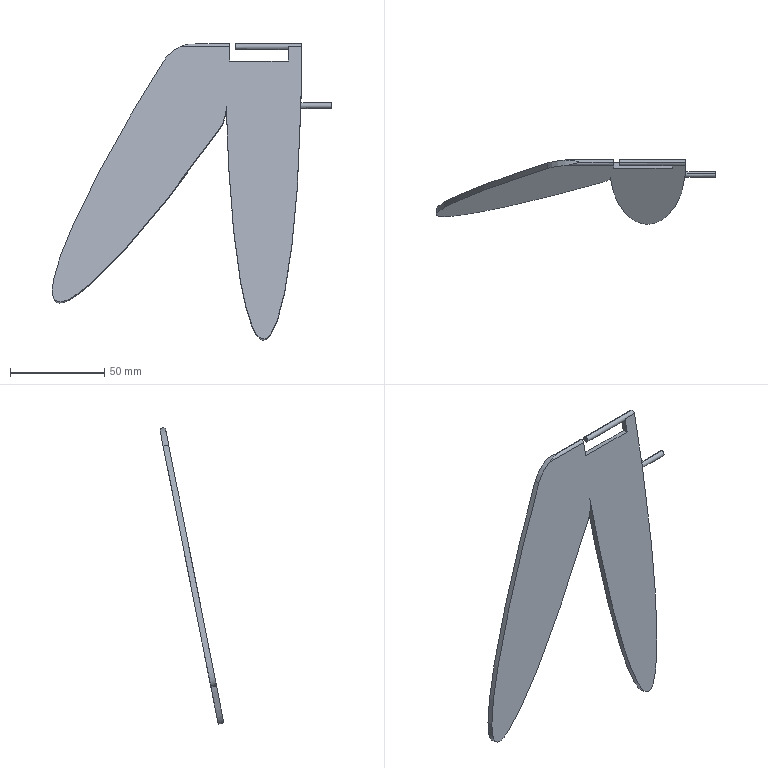Component | SolidWorks | 11-1 | 1 solid | 21 faces | box 147.82 x 33.71 x 156.77 mm | volume 30727 mm3 | cylinder 9 | plane 8 | spline 4 | commonest cylinder face diameters 3 x6 40 x3
STEP:
#1=CARTESIAN_POINT('',(1.359,2.476,-2.286));
#2=VERTEX_POINT('',#1);
#3=CARTESIAN_POINT('',(1.359,2.472,-2.304));
#4=VERTEX_POINT('',#3);
#5=CARTESIAN_POINT('',(0.5717,2.472,-2.304));
#6=DIRECTION('',(-0.,0.9809,-0.1945));
#7=DIRECTION('',(1.,0.,0.));
#8=AXIS2_PLACEMENT_3D('',#5,#6,#7);
#9=CIRCLE('',#8,0.7874);
#10=EDGE_CURVE('',#2,#4,#9,.T.);
#11=ORIENTED_EDGE('',*,*,#10,.T.);
#12=CARTESIAN_POINT('',(1.359,2.588,-2.327));
#13=VERTEX_POINT('',#12);
#14=CARTESIAN_POINT('',(1.359,2.472,-2.304));
#15=DIRECTION('',(-0.,0.9809,-0.1945));
#16=VECTOR('',#15,39.37);
#17=LINE('',#14,#16);
#18=EDGE_CURVE('',#4,#13,#17,.T.);
#19=ORIENTED_EDGE('',*,*,#18,.T.);
#20=CARTESIAN_POINT('',(1.359,2.592,-2.309));
#21=VERTEX_POINT('',#20);
#22=CARTESIAN_POINT('',(0.5717,2.588,-2.327));
#23=DIRECTION('',(-0.,0.9809,-0.1945));
#24=DIRECTION('',(1.,0.,0.));
#25=AXIS2_PLACEMENT_3D('',#22,#23,#24);
#26=CIRCLE('',#25,0.7874);
#27=EDGE_CURVE('',#21,#13,#26,.T.);
#28=ORIENTED_EDGE('',*,*,#27,.F.);
#29=CARTESIAN_POINT('',(1.359,2.476,-2.286));
#30=DIRECTION('',(-0.,0.9809,-0.1945));
#31=VECTOR('',#30,39.37);
#32=LINE('',#29,#31);
#33=EDGE_CURVE('',#2,#21,#32,.T.);
#34=ORIENTED_EDGE('',*,*,#33,.F.);
#35=EDGE_LOOP('',(#11,#19,#28,#34));
#36=FACE_OUTER_BOUND('',#35,.T.);
#37=CARTESIAN_POINT('',(0.5717,2.472,-2.304));
#38=DIRECTION('',(-0.,0.9809,-0.1945));
#39=DIRECTION('',(1.,0.,0.));
#40=AXIS2_PLACEMENT_3D('',#37,#38,#39);
#41=CYLINDRICAL_SURFACE('',#40,0.7874);
#42=ADVANCED_FACE('',(#36),#41,.T.);
#43=CARTESIAN_POINT('',(1.218,2.385,-2.745));
#44=VERTEX_POINT('',#43);
#45=CARTESIAN_POINT('',(-2.187,1.672,-6.337));
#46=VERTEX_POINT('',#45);
#47=CARTESIAN_POINT('',(1.218,2.385,-2.745));
#48=CARTESIAN_POINT('',(-0.5057,1.903,-5.172));
#49=CARTESIAN_POINT('',(-1.827,1.627,-6.566));
#50=CARTESIAN_POINT('',(-2.187,1.672,-6.337));
#51=(BOUNDED_CURVE()B_SPLINE_CURVE(3,(#47,#48,#49,#50),.UNSPECIFIED.,.F.,.T.)B_SPLINE_CURVE_WITH_KNOTS((4,4),(4.959,6.283),.UNSPECIFIED.)CURVE()GEOMETRIC_REPRESENTATION_ITEM()RATIONAL_B_SPLINE_CURVE((1.,0.8591,0.8591,1.))REPRESENTATION_ITEM(''));
#52=EDGE_CURVE('',#44,#46,#51,.T.);
#53=ORIENTED_EDGE('',*,*,#52,.T.);
#54=CARTESIAN_POINT('',(-2.187,1.788,-6.36));
#55=VERTEX_POINT('',#54);
#56=CARTESIAN_POINT('',(-2.187,1.672,-6.337));
#57=DIRECTION('',(-0.,0.9809,-0.1945));
#58=VECTOR('',#57,39.37);
#59=LINE('',#56,#58);
#60=EDGE_CURVE('',#46,#55,#59,.T.);
#61=ORIENTED_EDGE('',*,*,#60,.T.);
#62=CARTESIAN_POINT('',(1.218,2.501,-2.768));
#63=VERTEX_POINT('',#62);
#64=CARTESIAN_POINT('',(1.218,2.501,-2.768));
#65=CARTESIAN_POINT('',(-0.5057,2.019,-5.195));
#66=CARTESIAN_POINT('',(-1.827,1.743,-6.589));
#67=CARTESIAN_POINT('',(-2.187,1.788,-6.36));
#68=(BOUNDED_CURVE()B_SPLINE_CURVE(3,(#64,#65,#66,#67),.UNSPECIFIED.,.F.,.T.)B_SPLINE_CURVE_WITH_KNOTS((4,4),(4.959,6.283),.UNSPECIFIED.)CURVE()GEOMETRIC_REPRESENTATION_ITEM()RATIONAL_B_SPLINE_CURVE((1.,0.8591,0.8591,1.))REPRESENTATION_ITEM(''));
#69=EDGE_CURVE('',#63,#55,#68,.T.);
#70=ORIENTED_EDGE('',*,*,#69,.F.);
#71=CARTESIAN_POINT('',(1.218,2.385,-2.745));
#72=DIRECTION('',(-0.,0.9809,-0.1945));
#73=VECTOR('',#72,39.37);
#74=LINE('',#71,#73);
#75=EDGE_CURVE('',#44,#63,#74,.T.);
#76=ORIENTED_EDGE('',*,*,#75,.F.);
#77=EDGE_LOOP('',(#53,#61,#70,#76));
#78=FACE_OUTER_BOUND('',#77,.T.);
#79=CARTESIAN_POINT('',(1.218,2.385,-2.745));
#80=CARTESIAN_POINT('',(1.218,2.501,-2.768));
#81=CARTESIAN_POINT('',(-0.5057,1.903,-5.172));
#82=CARTESIAN_POINT('',(-0.5057,2.019,-5.195));
#83=CARTESIAN_POINT('',(-1.827,1.627,-6.566));
#84=CARTESIAN_POINT('',(-1.827,1.743,-6.589));
#85=CARTESIAN_POINT('',(-2.187,1.672,-6.337));
#86=CARTESIAN_POINT('',(-2.187,1.788,-6.36));
#87=(BOUNDED_SURFACE()B_SPLINE_SURFACE(3,1,((#79,#80),(#81,#82),(#83,#84),(#85,#86)),.UNSPECIFIED.,.F.,.F.,.T.)B_SPLINE_SURFACE_WITH_KNOTS((4,4),(2,2),(0.,1.),(0.,1.),.UNSPECIFIED.)GEOMETRIC_REPRESENTATION_ITEM()RATIONAL_B_SPLINE_SURFACE(((1.,1.),(0.8591,0.8591),(0.8591,0.8591),(1.,1.)))REPRESENTATION_ITEM('')SURFACE());
#88=ADVANCED_FACE('',(#78),#87,.T.);
#89=CARTESIAN_POINT('',(3.553,2.528,-2.328));
#90=VERTEX_POINT('',#89);
#91=CARTESIAN_POINT('',(3.553,2.551,-2.212));
#92=VERTEX_POINT('',#91);
#93=CARTESIAN_POINT('',(3.553,2.539,-2.27));
#94=DIRECTION('',(1.,0.,0.));
#95=DIRECTION('',(0.,-0.1945,-0.9809));
#96=AXIS2_PLACEMENT_3D('',#93,#94,#95);
#97=CIRCLE('',#96,0.05906);
#98=EDGE_CURVE('',#90,#92,#97,.T.);
#99=ORIENTED_EDGE('',*,*,#98,.F.);
#100=CARTESIAN_POINT('',(2.912,2.528,-2.328));
#101=VERTEX_POINT('',#100);
#102=CARTESIAN_POINT('',(3.553,2.528,-2.328));
#103=DIRECTION('',(-1.,-0.,-0.));
#104=VECTOR('',#103,39.37);
#105=LINE('',#102,#104);
#106=EDGE_CURVE('',#90,#101,#105,.T.);
#107=ORIENTED_EDGE('',*,*,#106,.T.);
#108=CARTESIAN_POINT('',(2.913,2.597,-2.282));
#109=VERTEX_POINT('',#108);
#110=CARTESIAN_POINT('',(2.913,2.597,-2.282));
#111=CARTESIAN_POINT('',(2.913,2.596,-2.289));
#112=CARTESIAN_POINT('',(2.913,2.592,-2.297));
#113=CARTESIAN_POINT('',(2.912,2.584,-2.309));
#114=CARTESIAN_POINT('',(2.912,2.578,-2.315));
#115=CARTESIAN_POINT('',(2.912,2.569,-2.322));
#116=CARTESIAN_POINT('',(2.912,2.565,-2.323));
#117=CARTESIAN_POINT('',(2.912,2.558,-2.326));
#118=CARTESIAN_POINT('',(2.912,2.554,-2.327));
#119=CARTESIAN_POINT('',(2.912,2.547,-2.329));
#120=CARTESIAN_POINT('',(2.912,2.543,-2.329));
#121=CARTESIAN_POINT('',(2.912,2.535,-2.329));
#122=CARTESIAN_POINT('',(2.912,2.531,-2.329));
#123=CARTESIAN_POINT('',(2.912,2.528,-2.328));
#124=B_SPLINE_CURVE_WITH_KNOTS('',3,(#110,#111,#112,#113,#114,#115,#116,#117,#118,#119,#120,#121,#122,#123),.UNSPECIFIED.,.F.,.F.,(4,2,2,2,2,2,4),(0.00469,0.005277,0.005863,0.006156,0.00645,0.006743,0.007036),.UNSPECIFIED.);
#125=EDGE_CURVE('',#109,#101,#124,.T.);
#126=ORIENTED_EDGE('',*,*,#125,.F.);
#127=CARTESIAN_POINT('',(2.914,2.551,-2.212));
#128=VERTEX_POINT('',#127);
#129=CARTESIAN_POINT('',(2.914,2.551,-2.212));
#130=CARTESIAN_POINT('',(2.914,2.554,-2.213));
#131=CARTESIAN_POINT('',(2.914,2.558,-2.214));
#132=CARTESIAN_POINT('',(2.914,2.565,-2.217));
#133=CARTESIAN_POINT('',(2.914,2.569,-2.219));
#134=CARTESIAN_POINT('',(2.914,2.575,-2.223));
#135=CARTESIAN_POINT('',(2.914,2.578,-2.226));
#136=CARTESIAN_POINT('',(2.914,2.584,-2.231));
#137=CARTESIAN_POINT('',(2.914,2.586,-2.234));
#138=CARTESIAN_POINT('',(2.914,2.592,-2.244));
#139=CARTESIAN_POINT('',(2.914,2.595,-2.251));
#140=CARTESIAN_POINT('',(2.914,2.598,-2.263));
#141=CARTESIAN_POINT('',(2.913,2.598,-2.266));
#142=CARTESIAN_POINT('',(2.913,2.598,-2.274));
#143=CARTESIAN_POINT('',(2.913,2.598,-2.278));
#144=CARTESIAN_POINT('',(2.913,2.597,-2.282));
#145=B_SPLINE_CURVE_WITH_KNOTS('',3,(#129,#130,#131,#132,#133,#134,#135,#136,#137,#138,#139,#140,#141,#142,#143,#144),.UNSPECIFIED.,.F.,.F.,(4,2,2,2,2,2,2,4),(0.002346,0.002639,0.002932,0.003225,0.003518,0.004104,0.004397,0.00469),.UNSPECIFIED.);
#146=EDGE_CURVE('',#128,#109,#145,.T.);
#147=ORIENTED_EDGE('',*,*,#146,.F.);
#148=CARTESIAN_POINT('',(3.553,2.551,-2.212));
#149=DIRECTION('',(-1.,-0.,-0.));
#150=VECTOR('',#149,39.37);
#151=LINE('',#148,#150);
#152=EDGE_CURVE('',#92,#128,#151,.T.);
#153=ORIENTED_EDGE('',*,*,#152,.F.);
#154=EDGE_LOOP('',(#99,#107,#126,#147,#153));
#155=FACE_OUTER_BOUND('',#154,.T.);
#156=CARTESIAN_POINT('',(3.553,2.539,-2.27));
#157=DIRECTION('',(-1.,-0.,-0.));
#158=DIRECTION('',(0.,0.1945,0.9809));
#159=AXIS2_PLACEMENT_3D('',#156,#157,#158);
#160=CYLINDRICAL_SURFACE('',#159,0.05906);
#161=ADVANCED_FACE('',(#155),#160,.T.);
#162=CARTESIAN_POINT('',(1.427,2.794,-0.9829));
#163=VERTEX_POINT('',#162);
#164=CARTESIAN_POINT('',(1.427,2.725,-1.029));
#165=VERTEX_POINT('',#164);
#166=CARTESIAN_POINT('',(1.427,2.783,-1.041));
#167=DIRECTION('',(1.,0.,0.));
#168=DIRECTION('',(0.,-0.1945,-0.9809));
#169=AXIS2_PLACEMENT_3D('',#166,#167,#168);
#170=CIRCLE('',#169,0.05906);
#171=EDGE_CURVE('',#163,#165,#170,.T.);
#172=ORIENTED_EDGE('',*,*,#171,.F.);
#173=CARTESIAN_POINT('',(0.7196,2.794,-0.9829));
#174=VERTEX_POINT('',#173);
#175=CARTESIAN_POINT('',(2.923,2.794,-0.9829));
#176=DIRECTION('',(-1.,-0.,-0.));
#177=VECTOR('',#176,39.37);
#178=LINE('',#175,#177);
#179=EDGE_CURVE('',#163,#174,#178,.T.);
#180=ORIENTED_EDGE('',*,*,#179,.T.);
#181=CARTESIAN_POINT('',(0.4204,2.725,-1.029));
#182=VERTEX_POINT('',#181);
#183=CARTESIAN_POINT('',(0.7196,2.794,-0.9829));
#184=CARTESIAN_POINT('',(0.7071,2.791,-0.9823));
#185=CARTESIAN_POINT('',(0.6944,2.788,-0.9819));
#186=CARTESIAN_POINT('',(0.6692,2.781,-0.9818));
#187=CARTESIAN_POINT('',(0.6567,2.777,-0.982));
#188=CARTESIAN_POINT('',(0.619,2.767,-0.9836));
#189=CARTESIAN_POINT('',(0.594,2.76,-0.986));
#190=CARTESIAN_POINT('',(0.544,2.747,-0.9934));
#191=CARTESIAN_POINT('',(0.5188,2.741,-0.9984));
#192=CARTESIAN_POINT('',(0.4693,2.731,-1.012));
#193=CARTESIAN_POINT('',(0.4448,2.727,-1.02));
#194=CARTESIAN_POINT('',(0.4204,2.725,-1.029));
#195=B_SPLINE_CURVE_WITH_KNOTS('',3,(#183,#184,#185,#186,#187,#188,#189,#190,#191,#192,#193,#194),.UNSPECIFIED.,.F.,.F.,(4,2,2,2,2,4),(-0.00002828,0.0009634,0.001955,0.003939,0.005922,0.007905),.UNSPECIFIED.);
#196=EDGE_CURVE('',#174,#182,#195,.T.);
#197=ORIENTED_EDGE('',*,*,#196,.T.);
#198=CARTESIAN_POINT('',(1.348,2.725,-1.029));
#199=DIRECTION('',(1.,0.,0.));
#200=VECTOR('',#199,39.37);
#201=LINE('',#198,#200);
#202=EDGE_CURVE('',#182,#165,#201,.T.);
#203=ORIENTED_EDGE('',*,*,#202,.T.);
#204=EDGE_LOOP('',(#172,#180,#197,#203));
#205=FACE_OUTER_BOUND('',#204,.T.);
#206=CARTESIAN_POINT('',(2.923,2.783,-1.041));
#207=DIRECTION('',(-1.,-0.,-0.));
#208=DIRECTION('',(0.,0.1945,0.9809));
#209=AXIS2_PLACEMENT_3D('',#206,#207,#208);
#210=CYLINDRICAL_SURFACE('',#209,0.05906);
#211=ADVANCED_FACE('',(#205),#210,.T.);
#212=CARTESIAN_POINT('',(2.648,2.771,-1.099));
#213=VERTEX_POINT('',#212);
#214=CARTESIAN_POINT('',(2.648,2.841,-1.052));
#215=VERTEX_POINT('',#214);
#216=CARTESIAN_POINT('',(2.648,2.783,-1.041));
#217=DIRECTION('',(1.,0.,0.));
#218=DIRECTION('',(0.,0.1945,0.9809));
#219=AXIS2_PLACEMENT_3D('',#216,#217,#218);
#220=CIRCLE('',#219,0.05906);
#221=EDGE_CURVE('',#213,#215,#220,.T.);
#222=ORIENTED_EDGE('',*,*,#221,.F.);
#223=CARTESIAN_POINT('',(1.545,2.771,-1.099));
#224=VERTEX_POINT('',#223);
#225=CARTESIAN_POINT('',(2.923,2.771,-1.099));
#226=DIRECTION('',(-1.,-0.,-0.));
#227=VECTOR('',#226,39.37);
#228=LINE('',#225,#227);
#229=EDGE_CURVE('',#213,#224,#228,.T.);
#230=ORIENTED_EDGE('',*,*,#229,.T.);
#231=CARTESIAN_POINT('',(1.545,2.794,-0.9829));
#232=VERTEX_POINT('',#231);
#233=CARTESIAN_POINT('',(1.545,2.783,-1.041));
#234=DIRECTION('',(-1.,-0.,-0.));
#235=DIRECTION('',(0.,0.1945,0.9809));
#236=AXIS2_PLACEMENT_3D('',#233,#234,#235);
#237=CIRCLE('',#236,0.05906);
#238=EDGE_CURVE('',#232,#224,#237,.T.);
#239=ORIENTED_EDGE('',*,*,#238,.F.);
#240=CARTESIAN_POINT('',(2.923,2.794,-0.9829));
#241=VERTEX_POINT('',#240);
#242=CARTESIAN_POINT('',(2.923,2.794,-0.9829));
#243=DIRECTION('',(-1.,-0.,-0.));
#244=VECTOR('',#243,39.37);
#245=LINE('',#242,#244);
#246=EDGE_CURVE('',#241,#232,#245,.T.);
#247=ORIENTED_EDGE('',*,*,#246,.F.);
#248=CARTESIAN_POINT('',(2.923,2.841,-1.052));
#249=VERTEX_POINT('',#248);
#250=CARTESIAN_POINT('',(2.923,2.783,-1.041));
#251=DIRECTION('',(1.,0.,0.));
#252=DIRECTION('',(0.,-0.1945,-0.9809));
#253=AXIS2_PLACEMENT_3D('',#250,#251,#252);
#254=CIRCLE('',#253,0.05906);
#255=EDGE_CURVE('',#249,#241,#254,.T.);
#256=ORIENTED_EDGE('',*,*,#255,.F.);
#257=CARTESIAN_POINT('',(2.844,2.841,-1.052));
#258=DIRECTION('',(1.,0.,0.));
#259=VECTOR('',#258,39.37);
#260=LINE('',#257,#259);
#261=EDGE_CURVE('',#215,#249,#260,.T.);
#262=ORIENTED_EDGE('',*,*,#261,.F.);
#263=EDGE_LOOP('',(#222,#230,#239,#247,#256,#262));
#264=FACE_OUTER_BOUND('',#263,.T.);
#265=CARTESIAN_POINT('',(2.923,2.783,-1.041));
#266=DIRECTION('',(-1.,-0.,-0.));
#267=DIRECTION('',(0.,0.1945,0.9809));
#268=AXIS2_PLACEMENT_3D('',#265,#266,#267);
#269=CYLINDRICAL_SURFACE('',#268,0.05906);
#270=ADVANCED_FACE('',(#264),#269,.T.);
#271=ORIENTED_EDGE('',*,*,#229,.F.);
#272=CARTESIAN_POINT('',(2.648,2.725,-1.029));
#273=VERTEX_POINT('',#272);
#274=CARTESIAN_POINT('',(2.648,2.783,-1.041));
#275=DIRECTION('',(1.,0.,0.));
#276=DIRECTION('',(0.,0.1945,0.9809));
#277=AXIS2_PLACEMENT_3D('',#274,#275,#276);
#278=CIRCLE('',#277,0.05906);
#279=EDGE_CURVE('',#273,#213,#278,.T.);
#280=ORIENTED_EDGE('',*,*,#279,.F.);
#281=CARTESIAN_POINT('',(2.923,2.725,-1.029));
#282=VERTEX_POINT('',#281);
#283=CARTESIAN_POINT('',(2.844,2.725,-1.029));
#284=DIRECTION('',(1.,0.,0.));
#285=VECTOR('',#284,39.37);
#286=LINE('',#283,#285);
#287=EDGE_CURVE('',#273,#282,#286,.T.);
#288=ORIENTED_EDGE('',*,*,#287,.T.);
#289=CARTESIAN_POINT('',(2.923,2.783,-1.041));
#290=DIRECTION('',(1.,0.,0.));
#291=DIRECTION('',(0.,-0.1945,-0.9809));
#292=AXIS2_PLACEMENT_3D('',#289,#290,#291);
#293=CIRCLE('',#292,0.05906);
#294=EDGE_CURVE('',#241,#282,#293,.T.);
#295=ORIENTED_EDGE('',*,*,#294,.F.);
#296=ORIENTED_EDGE('',*,*,#246,.T.);
#297=CARTESIAN_POINT('',(1.545,2.783,-1.041));
#298=DIRECTION('',(-1.,-0.,-0.));
#299=DIRECTION('',(0.,0.1945,0.9809));
#300=AXIS2_PLACEMENT_3D('',#297,#298,#299);
#301=CIRCLE('',#300,0.05906);
#302=EDGE_CURVE('',#224,#232,#301,.T.);
#303=ORIENTED_EDGE('',*,*,#302,.F.);
#304=EDGE_LOOP('',(#271,#280,#288,#295,#296,#303));
#305=FACE_OUTER_BOUND('',#304,.T.);
#306=CARTESIAN_POINT('',(2.923,2.783,-1.041));
#307=DIRECTION('',(-1.,-0.,-0.));
#308=DIRECTION('',(0.,0.1945,0.9809));
#309=AXIS2_PLACEMENT_3D('',#306,#307,#308);
#310=CYLINDRICAL_SURFACE('',#309,0.05906);
#311=ADVANCED_FACE('',(#305),#310,.T.);
#312=ORIENTED_EDGE('',*,*,#179,.F.);
#313=CARTESIAN_POINT('',(1.427,2.841,-1.052));
#314=VERTEX_POINT('',#313);
#315=CARTESIAN_POINT('',(1.427,2.783,-1.041));
#316=DIRECTION('',(1.,0.,0.));
#317=DIRECTION('',(0.,-0.1945,-0.9809));
#318=AXIS2_PLACEMENT_3D('',#315,#316,#317);
#319=CIRCLE('',#318,0.05906);
#320=EDGE_CURVE('',#314,#163,#319,.T.);
#321=ORIENTED_EDGE('',*,*,#320,.F.);
#322=CARTESIAN_POINT('',(0.4204,2.841,-1.052));
#323=VERTEX_POINT('',#322);
#324=CARTESIAN_POINT('',(1.348,2.841,-1.052));
#325=DIRECTION('',(1.,0.,0.));
#326=VECTOR('',#325,39.37);
#327=LINE('',#324,#326);
#328=EDGE_CURVE('',#323,#314,#327,.T.);
#329=ORIENTED_EDGE('',*,*,#328,.F.);
#330=CARTESIAN_POINT('',(0.4204,2.841,-1.052));
#331=CARTESIAN_POINT('',(0.4448,2.843,-1.043));
#332=CARTESIAN_POINT('',(0.4693,2.842,-1.034));
#333=CARTESIAN_POINT('',(0.5188,2.838,-1.018));
#334=CARTESIAN_POINT('',(0.544,2.834,-1.011));
#335=CARTESIAN_POINT('',(0.594,2.825,-0.9989));
#336=CARTESIAN_POINT('',(0.619,2.82,-0.9941));
#337=CARTESIAN_POINT('',(0.6566,2.811,-0.9886));
#338=CARTESIAN_POINT('',(0.6692,2.808,-0.9871));
#339=CARTESIAN_POINT('',(0.6944,2.801,-0.9846));
#340=CARTESIAN_POINT('',(0.707,2.798,-0.9836));
#341=CARTESIAN_POINT('',(0.7196,2.794,-0.9829));
#342=B_SPLINE_CURVE_WITH_KNOTS('',3,(#330,#331,#332,#333,#334,#335,#336,#337,#338,#339,#340,#341),.UNSPECIFIED.,.F.,.F.,(4,2,2,2,2,4),(0.,0.001988,0.003977,0.005965,0.00696,0.007954),.UNSPECIFIED.);
#343=EDGE_CURVE('',#323,#174,#342,.T.);
#344=ORIENTED_EDGE('',*,*,#343,.T.);
#345=EDGE_LOOP('',(#312,#321,#329,#344));
#346=FACE_OUTER_BOUND('',#345,.T.);
#347=CARTESIAN_POINT('',(2.923,2.783,-1.041));
#348=DIRECTION('',(-1.,-0.,-0.));
#349=DIRECTION('',(0.,0.1945,0.9809));
#350=AXIS2_PLACEMENT_3D('',#347,#348,#349);
#351=CYLINDRICAL_SURFACE('',#350,0.05906);
#352=ADVANCED_FACE('',(#346),#351,.T.);
#353=CARTESIAN_POINT('',(2.648,2.78,-1.361));
#354=VERTEX_POINT('',#353);
#355=CARTESIAN_POINT('',(2.648,2.841,-1.052));
#356=DIRECTION('',(0.,-0.1945,-0.9809));
#357=VECTOR('',#356,39.37);
#358=LINE('',#355,#357);
#359=EDGE_CURVE('',#215,#354,#358,.T.);
#360=ORIENTED_EDGE('',*,*,#359,.F.);
#361=ORIENTED_EDGE('',*,*,#261,.T.);
#362=CARTESIAN_POINT('',(2.923,2.78,-1.361));
#363=VERTEX_POINT('',#362);
#364=CARTESIAN_POINT('',(2.923,2.841,-1.052));
#365=DIRECTION('',(0.,-0.1945,-0.9809));
#366=VECTOR('',#365,39.37);
#367=LINE('',#364,#366);
#368=EDGE_CURVE('',#249,#363,#367,.T.);
#369=ORIENTED_EDGE('',*,*,#368,.T.);
#370=CARTESIAN_POINT('',(2.923,2.78,-1.361));
#371=CARTESIAN_POINT('',(2.923,2.718,-1.67));
#372=CARTESIAN_POINT('',(2.92,2.657,-1.977));
#373=CARTESIAN_POINT('',(2.913,2.597,-2.282));
#374=(BOUNDED_CURVE()B_SPLINE_CURVE(3,(#370,#371,#372,#373),.UNSPECIFIED.,.F.,.T.)B_SPLINE_CURVE_WITH_KNOTS((4,4),(1.571,1.73),.UNSPECIFIED.)CURVE()GEOMETRIC_REPRESENTATION_ITEM()RATIONAL_B_SPLINE_CURVE((1.,0.9979,0.9979,1.))REPRESENTATION_ITEM(''));
#375=EDGE_CURVE('',#363,#109,#374,.T.);
#376=ORIENTED_EDGE('',*,*,#375,.T.);
#377=CARTESIAN_POINT('',(2.913,2.597,-2.282));
#378=CARTESIAN_POINT('',(2.726,0.9043,-10.817));
#379=CARTESIAN_POINT('',(1.551,0.9002,-10.838));
#380=CARTESIAN_POINT('',(1.359,2.592,-2.309));
#381=(BOUNDED_CURVE()B_SPLINE_CURVE(3,(#377,#378,#379,#380),.UNSPECIFIED.,.F.,.T.)B_SPLINE_CURVE_WITH_KNOTS((4,4),(1.73,4.548),.UNSPECIFIED.)CURVE()GEOMETRIC_REPRESENTATION_ITEM()RATIONAL_B_SPLINE_CURVE((1.,0.4409,0.4409,1.))REPRESENTATION_ITEM(''));
#382=EDGE_CURVE('',#109,#21,#381,.T.);
#383=ORIENTED_EDGE('',*,*,#382,.T.);
#384=ORIENTED_EDGE('',*,*,#27,.T.);
#385=CARTESIAN_POINT('',(0.5717,2.588,-2.327));
#386=DIRECTION('',(-0.,0.9809,-0.1945));
#387=DIRECTION('',(1.,0.,0.));
#388=AXIS2_PLACEMENT_3D('',#385,#386,#387);
#389=CIRCLE('',#388,0.7874);
#390=EDGE_CURVE('',#13,#63,#389,.T.);
#391=ORIENTED_EDGE('',*,*,#390,.T.);
#392=ORIENTED_EDGE('',*,*,#69,.T.);
#393=CARTESIAN_POINT('',(0.0491,2.779,-1.362));
#394=VERTEX_POINT('',#393);
#395=CARTESIAN_POINT('',(-2.187,1.788,-6.36));
#396=CARTESIAN_POINT('',(-2.576,1.837,-6.114));
#397=CARTESIAN_POINT('',(-1.689,2.23,-4.131));
#398=CARTESIAN_POINT('',(0.0491,2.779,-1.362));
#399=(BOUNDED_CURVE()B_SPLINE_CURVE(3,(#395,#396,#397,#398),.UNSPECIFIED.,.F.,.T.)B_SPLINE_CURVE_WITH_KNOTS((4,4),(0.,1.414),.UNSPECIFIED.)CURVE()GEOMETRIC_REPRESENTATION_ITEM()RATIONAL_B_SPLINE_CURVE((1.,0.8403,0.8403,1.))REPRESENTATION_ITEM(''));
#400=EDGE_CURVE('',#55,#394,#399,.T.);
#401=ORIENTED_EDGE('',*,*,#400,.T.);
#402=CARTESIAN_POINT('',(0.7196,2.699,-1.767));
#403=DIRECTION('',(-0.,0.9809,-0.1945));
#404=DIRECTION('',(-1.,0.,-0.));
#405=AXIS2_PLACEMENT_3D('',#402,#403,#404);
#406=CIRCLE('',#405,0.7874);
#407=EDGE_CURVE('',#394,#323,#406,.T.);
#408=ORIENTED_EDGE('',*,*,#407,.T.);
#409=ORIENTED_EDGE('',*,*,#328,.T.);
#410=CARTESIAN_POINT('',(1.427,2.78,-1.361));
#411=VERTEX_POINT('',#410);
#412=CARTESIAN_POINT('',(1.427,2.829,-1.11));
#413=DIRECTION('',(0.,-0.1945,-0.9809));
#414=VECTOR('',#413,39.37);
#415=LINE('',#412,#414);
#416=EDGE_CURVE('',#314,#411,#415,.T.);
#417=ORIENTED_EDGE('',*,*,#416,.T.);
#418=CARTESIAN_POINT('',(1.348,2.78,-1.361));
#419=DIRECTION('',(1.,0.,0.));
#420=VECTOR('',#419,39.37);
#421=LINE('',#418,#420);
#422=EDGE_CURVE('',#411,#354,#421,.T.);
#423=ORIENTED_EDGE('',*,*,#422,.T.);
#424=EDGE_LOOP('',(#360,#361,#369,#376,#383,#384,#391,#392,#401,#408,#409,#417,#423));
#425=FACE_OUTER_BOUND('',#424,.T.);
#426=CARTESIAN_POINT('',(1.348,2.841,-1.052));
#427=DIRECTION('',(0.,-0.9809,0.1945));
#428=DIRECTION('',(-1.,-0.,-0.));
#429=AXIS2_PLACEMENT_3D('',#426,#427,#428);
#430=PLANE('',#429);
#431=ADVANCED_FACE('',(#425),#430,.F.);
#432=ORIENTED_EDGE('',*,*,#287,.F.);
#433=CARTESIAN_POINT('',(2.648,2.664,-1.338));
#434=VERTEX_POINT('',#433);
#435=CARTESIAN_POINT('',(2.648,2.664,-1.338));
#436=DIRECTION('',(-0.,0.1945,0.9809));
#437=VECTOR('',#436,39.37);
#438=LINE('',#435,#437);
#439=EDGE_CURVE('',#434,#273,#438,.T.);
#440=ORIENTED_EDGE('',*,*,#439,.F.);
#441=CARTESIAN_POINT('',(1.427,2.664,-1.338));
#442=VERTEX_POINT('',#441);
#443=CARTESIAN_POINT('',(1.348,2.664,-1.338));
#444=DIRECTION('',(1.,0.,0.));
#445=VECTOR('',#444,39.37);
#446=LINE('',#443,#445);
#447=EDGE_CURVE('',#442,#434,#446,.T.);
#448=ORIENTED_EDGE('',*,*,#447,.F.);
#449=CARTESIAN_POINT('',(1.427,2.664,-1.338));
#450=DIRECTION('',(0.,-0.1945,-0.9809));
#451=VECTOR('',#450,39.37);
#452=LINE('',#449,#451);
#453=EDGE_CURVE('',#165,#442,#452,.T.);
#454=ORIENTED_EDGE('',*,*,#453,.F.);
#455=ORIENTED_EDGE('',*,*,#202,.F.);
#456=CARTESIAN_POINT('',(0.0491,2.664,-1.339));
#457=VERTEX_POINT('',#456);
#458=CARTESIAN_POINT('',(0.7196,2.583,-1.744));
#459=DIRECTION('',(-0.,0.9809,-0.1945));
#460=DIRECTION('',(-1.,0.,-0.));
#461=AXIS2_PLACEMENT_3D('',#458,#459,#460);
#462=CIRCLE('',#461,0.7874);
#463=EDGE_CURVE('',#457,#182,#462,.T.);
#464=ORIENTED_EDGE('',*,*,#463,.F.);
#465=CARTESIAN_POINT('',(-2.187,1.672,-6.337));
#466=CARTESIAN_POINT('',(-2.576,1.721,-6.091));
#467=CARTESIAN_POINT('',(-1.689,2.114,-4.108));
#468=CARTESIAN_POINT('',(0.0491,2.664,-1.339));
#469=(BOUNDED_CURVE()B_SPLINE_CURVE(3,(#465,#466,#467,#468),.UNSPECIFIED.,.F.,.T.)B_SPLINE_CURVE_WITH_KNOTS((4,4),(0.,1.414),.UNSPECIFIED.)CURVE()GEOMETRIC_REPRESENTATION_ITEM()RATIONAL_B_SPLINE_CURVE((1.,0.8403,0.8403,1.))REPRESENTATION_ITEM(''));
#470=EDGE_CURVE('',#46,#457,#469,.T.);
#471=ORIENTED_EDGE('',*,*,#470,.F.);
#472=ORIENTED_EDGE('',*,*,#52,.F.);
#473=CARTESIAN_POINT('',(0.5717,2.472,-2.304));
#474=DIRECTION('',(-0.,0.9809,-0.1945));
#475=DIRECTION('',(1.,0.,0.));
#476=AXIS2_PLACEMENT_3D('',#473,#474,#475);
#477=CIRCLE('',#476,0.7874);
#478=EDGE_CURVE('',#4,#44,#477,.T.);
#479=ORIENTED_EDGE('',*,*,#478,.F.);
#480=ORIENTED_EDGE('',*,*,#10,.F.);
#481=CARTESIAN_POINT('',(2.913,2.481,-2.259));
#482=VERTEX_POINT('',#481);
#483=CARTESIAN_POINT('',(2.913,2.481,-2.259));
#484=CARTESIAN_POINT('',(2.726,0.7884,-10.794));
#485=CARTESIAN_POINT('',(1.551,0.7843,-10.815));
#486=CARTESIAN_POINT('',(1.359,2.476,-2.286));
#487=(BOUNDED_CURVE()B_SPLINE_CURVE(3,(#483,#484,#485,#486),.UNSPECIFIED.,.F.,.T.)B_SPLINE_CURVE_WITH_KNOTS((4,4),(1.73,4.548),.UNSPECIFIED.)CURVE()GEOMETRIC_REPRESENTATION_ITEM()RATIONAL_B_SPLINE_CURVE((1.,0.4409,0.4409,1.))REPRESENTATION_ITEM(''));
#488=EDGE_CURVE('',#482,#2,#487,.T.);
#489=ORIENTED_EDGE('',*,*,#488,.F.);
#490=CARTESIAN_POINT('',(2.923,2.664,-1.338));
#491=VERTEX_POINT('',#490);
#492=CARTESIAN_POINT('',(2.923,2.664,-1.338));
#493=CARTESIAN_POINT('',(2.923,2.603,-1.647));
#494=CARTESIAN_POINT('',(2.92,2.542,-1.954));
#495=CARTESIAN_POINT('',(2.913,2.481,-2.259));
#496=(BOUNDED_CURVE()B_SPLINE_CURVE(3,(#492,#493,#494,#495),.UNSPECIFIED.,.F.,.T.)B_SPLINE_CURVE_WITH_KNOTS((4,4),(1.571,1.73),.UNSPECIFIED.)CURVE()GEOMETRIC_REPRESENTATION_ITEM()RATIONAL_B_SPLINE_CURVE((1.,0.9979,0.9979,1.))REPRESENTATION_ITEM(''));
#497=EDGE_CURVE('',#491,#482,#496,.T.);
#498=ORIENTED_EDGE('',*,*,#497,.F.);
#499=CARTESIAN_POINT('',(2.923,2.725,-1.029));
#500=DIRECTION('',(0.,-0.1945,-0.9809));
#501=VECTOR('',#500,39.37);
#502=LINE('',#499,#501);
#503=EDGE_CURVE('',#282,#491,#502,.T.);
#504=ORIENTED_EDGE('',*,*,#503,.F.);
#505=EDGE_LOOP('',(#432,#440,#448,#454,#455,#464,#471,#472,#479,#480,#489,#498,#504));
#506=FACE_OUTER_BOUND('',#505,.T.);
#507=CARTESIAN_POINT('',(1.348,2.725,-1.029));
#508=DIRECTION('',(0.,-0.9809,0.1945));
#509=DIRECTION('',(-1.,-0.,-0.));
#510=AXIS2_PLACEMENT_3D('',#507,#508,#509);
#511=PLANE('',#510);
#512=ADVANCED_FACE('',(#506),#511,.T.);
#513=ORIENTED_EDGE('',*,*,#488,.T.);
#514=ORIENTED_EDGE('',*,*,#33,.T.);
#515=ORIENTED_EDGE('',*,*,#382,.F.);
#516=ORIENTED_EDGE('',*,*,#125,.T.);
#517=CARTESIAN_POINT('',(2.912,2.528,-2.328));
#518=CARTESIAN_POINT('',(2.912,2.52,-2.327));
#519=CARTESIAN_POINT('',(2.912,2.513,-2.324));
#520=CARTESIAN_POINT('',(2.912,2.503,-2.317));
#521=CARTESIAN_POINT('',(2.912,2.5,-2.315));
#522=CARTESIAN_POINT('',(2.912,2.495,-2.309));
#523=CARTESIAN_POINT('',(2.912,2.492,-2.306));
#524=CARTESIAN_POINT('',(2.912,2.486,-2.297));
#525=CARTESIAN_POINT('',(2.912,2.483,-2.289));
#526=CARTESIAN_POINT('',(2.913,2.48,-2.274));
#527=CARTESIAN_POINT('',(2.913,2.48,-2.266));
#528=CARTESIAN_POINT('',(2.913,2.481,-2.259));
#529=B_SPLINE_CURVE_WITH_KNOTS('',3,(#517,#518,#519,#520,#521,#522,#523,#524,#525,#526,#527,#528),.UNSPECIFIED.,.F.,.F.,(4,2,2,2,2,4),(0.007036,0.007622,0.007915,0.008208,0.008794,0.009379),.UNSPECIFIED.);
#530=EDGE_CURVE('',#101,#482,#529,.T.);
#531=ORIENTED_EDGE('',*,*,#530,.T.);
#532=EDGE_LOOP('',(#513,#514,#515,#516,#531));
#533=FACE_OUTER_BOUND('',#532,.T.);
#534=CARTESIAN_POINT('',(2.915,2.5,-2.162));
#535=CARTESIAN_POINT('',(2.915,2.616,-2.185));
#536=CARTESIAN_POINT('',(2.746,0.7793,-10.84));
#537=CARTESIAN_POINT('',(2.746,0.8951,-10.863));
#538=CARTESIAN_POINT('',(1.554,0.7604,-10.936));
#539=CARTESIAN_POINT('',(1.554,0.8762,-10.958));
#540=CARTESIAN_POINT('',(1.359,2.476,-2.286));
#541=CARTESIAN_POINT('',(1.359,2.592,-2.309));
#542=(BOUNDED_SURFACE()B_SPLINE_SURFACE(3,1,((#534,#535),(#536,#537),(#538,#539),(#540,#541)),.UNSPECIFIED.,.F.,.F.,.T.)B_SPLINE_SURFACE_WITH_KNOTS((4,4),(2,2),(0.,1.),(0.,1.),.UNSPECIFIED.)GEOMETRIC_REPRESENTATION_ITEM()RATIONAL_B_SPLINE_SURFACE(((1.,1.),(0.4353,0.4353),(0.4353,0.4353),(1.,1.)))REPRESENTATION_ITEM('')SURFACE());
#543=ADVANCED_FACE('',(#533),#542,.T.);
#544=ORIENTED_EDGE('',*,*,#497,.T.);
#545=CARTESIAN_POINT('',(2.913,2.481,-2.259));
#546=CARTESIAN_POINT('',(2.913,2.482,-2.255));
#547=CARTESIAN_POINT('',(2.913,2.483,-2.251));
#548=CARTESIAN_POINT('',(2.913,2.486,-2.244));
#549=CARTESIAN_POINT('',(2.914,2.488,-2.241));
#550=CARTESIAN_POINT('',(2.914,2.492,-2.234));
#551=CARTESIAN_POINT('',(2.914,2.495,-2.231));
#552=CARTESIAN_POINT('',(2.914,2.5,-2.226));
#553=CARTESIAN_POINT('',(2.914,2.503,-2.223));
#554=CARTESIAN_POINT('',(2.914,2.513,-2.217));
#555=CARTESIAN_POINT('',(2.914,2.52,-2.214));
#556=CARTESIAN_POINT('',(2.914,2.535,-2.211));
#557=CARTESIAN_POINT('',(2.914,2.543,-2.211));
#558=CARTESIAN_POINT('',(2.914,2.551,-2.212));
#559=B_SPLINE_CURVE_WITH_KNOTS('',3,(#545,#546,#547,#548,#549,#550,#551,#552,#553,#554,#555,#556,#557,#558),.UNSPECIFIED.,.F.,.F.,(4,2,2,2,2,2,4),(0.,0.0002932,0.0005864,0.0008796,0.001173,0.001759,0.002346),.UNSPECIFIED.);
#560=EDGE_CURVE('',#482,#128,#559,.T.);
#561=ORIENTED_EDGE('',*,*,#560,.T.);
#562=ORIENTED_EDGE('',*,*,#146,.T.);
#563=ORIENTED_EDGE('',*,*,#375,.F.);
#564=CARTESIAN_POINT('',(2.923,2.78,-1.361));
#565=DIRECTION('',(0.,-0.9809,0.1945));
#566=VECTOR('',#565,39.37);
#567=LINE('',#564,#566);
#568=EDGE_CURVE('',#363,#491,#567,.T.);
#569=ORIENTED_EDGE('',*,*,#568,.T.);
#570=EDGE_LOOP('',(#544,#561,#562,#563,#569));
#571=FACE_OUTER_BOUND('',#570,.T.);
#572=CARTESIAN_POINT('',(2.923,2.664,-1.338));
#573=CARTESIAN_POINT('',(2.923,2.78,-1.361));
#574=CARTESIAN_POINT('',(2.923,2.602,-1.649));
#575=CARTESIAN_POINT('',(2.923,2.718,-1.672));
#576=CARTESIAN_POINT('',(2.92,2.541,-1.958));
#577=CARTESIAN_POINT('',(2.92,2.657,-1.981));
#578=CARTESIAN_POINT('',(2.913,2.48,-2.264));
#579=CARTESIAN_POINT('',(2.913,2.596,-2.287));
#580=(BOUNDED_SURFACE()B_SPLINE_SURFACE(3,1,((#572,#573),(#574,#575),(#576,#577),(#578,#579)),.UNSPECIFIED.,.F.,.F.,.T.)B_SPLINE_SURFACE_WITH_KNOTS((4,4),(2,2),(0.,1.),(0.,1.),.UNSPECIFIED.)GEOMETRIC_REPRESENTATION_ITEM()RATIONAL_B_SPLINE_SURFACE(((1.,1.),(0.9979,0.9979),(0.9979,0.9979),(1.,1.)))REPRESENTATION_ITEM('')SURFACE());
#581=ADVANCED_FACE('',(#571),#580,.T.);
#582=ORIENTED_EDGE('',*,*,#255,.T.);
#583=ORIENTED_EDGE('',*,*,#294,.T.);
#584=ORIENTED_EDGE('',*,*,#503,.T.);
#585=ORIENTED_EDGE('',*,*,#568,.F.);
#586=ORIENTED_EDGE('',*,*,#368,.F.);
#587=EDGE_LOOP('',(#582,#583,#584,#585,#586));
#588=FACE_OUTER_BOUND('',#587,.T.);
#589=CARTESIAN_POINT('',(2.923,2.783,-1.041));
#590=DIRECTION('',(1.,0.,0.));
#591=DIRECTION('',(0.,-0.1945,-0.9809));
#592=AXIS2_PLACEMENT_3D('',#589,#590,#591);
#593=PLANE('',#592);
#594=ADVANCED_FACE('',(#588),#593,.T.);
#595=ORIENTED_EDGE('',*,*,#416,.F.);
#596=ORIENTED_EDGE('',*,*,#320,.T.);
#597=ORIENTED_EDGE('',*,*,#171,.T.);
#598=ORIENTED_EDGE('',*,*,#453,.T.);
#599=CARTESIAN_POINT('',(1.427,2.78,-1.361));
#600=DIRECTION('',(0.,-0.9809,0.1945));
#601=VECTOR('',#600,39.37);
#602=LINE('',#599,#601);
#603=EDGE_CURVE('',#411,#442,#602,.T.);
#604=ORIENTED_EDGE('',*,*,#603,.F.);
#605=EDGE_LOOP('',(#595,#596,#597,#598,#604));
#606=FACE_OUTER_BOUND('',#605,.T.);
#607=CARTESIAN_POINT('',(1.427,2.78,-1.361));
#608=DIRECTION('',(-1.,-0.,-0.));
#609=DIRECTION('',(-0.,0.1945,0.9809));
#610=AXIS2_PLACEMENT_3D('',#607,#608,#609);
#611=PLANE('',#610);
#612=ADVANCED_FACE('',(#606),#611,.F.);
#613=CARTESIAN_POINT('',(2.648,2.78,-1.361));
#614=DIRECTION('',(0.,-0.9809,0.1945));
#615=VECTOR('',#614,39.37);
#616=LINE('',#613,#615);
#617=EDGE_CURVE('',#354,#434,#616,.T.);
#618=ORIENTED_EDGE('',*,*,#617,.F.);
#619=ORIENTED_EDGE('',*,*,#422,.F.);
#620=ORIENTED_EDGE('',*,*,#603,.T.);
#621=ORIENTED_EDGE('',*,*,#447,.T.);
#622=EDGE_LOOP('',(#618,#619,#620,#621));
#623=FACE_OUTER_BOUND('',#622,.T.);
#624=CARTESIAN_POINT('',(1.348,2.664,-1.338));
#625=DIRECTION('',(-0.,0.1945,0.9809));
#626=DIRECTION('',(1.,0.,0.));
#627=AXIS2_PLACEMENT_3D('',#624,#625,#626);
#628=PLANE('',#627);
#629=ADVANCED_FACE('',(#623),#628,.T.);
#630=ORIENTED_EDGE('',*,*,#106,.F.);
#631=CARTESIAN_POINT('',(3.553,2.539,-2.27));
#632=DIRECTION('',(1.,0.,0.));
#633=DIRECTION('',(0.,-0.1945,-0.9809));
#634=AXIS2_PLACEMENT_3D('',#631,#632,#633);
#635=CIRCLE('',#634,0.05906);
#636=EDGE_CURVE('',#92,#90,#635,.T.);
#637=ORIENTED_EDGE('',*,*,#636,.F.);
#638=ORIENTED_EDGE('',*,*,#152,.T.);
#639=ORIENTED_EDGE('',*,*,#560,.F.);
#640=ORIENTED_EDGE('',*,*,#530,.F.);
#641=EDGE_LOOP('',(#630,#637,#638,#639,#640));
#642=FACE_OUTER_BOUND('',#641,.T.);
#643=CARTESIAN_POINT('',(3.553,2.539,-2.27));
#644=DIRECTION('',(-1.,-0.,-0.));
#645=DIRECTION('',(0.,0.1945,0.9809));
#646=AXIS2_PLACEMENT_3D('',#643,#644,#645);
#647=CYLINDRICAL_SURFACE('',#646,0.05906);
#648=ADVANCED_FACE('',(#642),#647,.T.);
#649=ORIENTED_EDGE('',*,*,#636,.T.);
#650=ORIENTED_EDGE('',*,*,#98,.T.);
#651=EDGE_LOOP('',(#649,#650));
#652=FACE_OUTER_BOUND('',#651,.T.);
#653=CARTESIAN_POINT('',(3.553,2.539,-2.27));
#654=DIRECTION('',(1.,0.,0.));
#655=DIRECTION('',(0.,-0.1945,-0.9809));
#656=AXIS2_PLACEMENT_3D('',#653,#654,#655);
#657=PLANE('',#656);
#658=ADVANCED_FACE('',(#652),#657,.T.);
#659=ORIENTED_EDGE('',*,*,#343,.F.);
#660=ORIENTED_EDGE('',*,*,#407,.F.);
#661=CARTESIAN_POINT('',(0.0491,2.664,-1.339));
#662=DIRECTION('',(-0.,0.9809,-0.1945));
#663=VECTOR('',#662,39.37);
#664=LINE('',#661,#663);
#665=EDGE_CURVE('',#457,#394,#664,.T.);
#666=ORIENTED_EDGE('',*,*,#665,.F.);
#667=ORIENTED_EDGE('',*,*,#463,.T.);
#668=ORIENTED_EDGE('',*,*,#196,.F.);
#669=EDGE_LOOP('',(#659,#660,#666,#667,#668));
#670=FACE_OUTER_BOUND('',#669,.T.);
#671=CARTESIAN_POINT('',(0.7196,2.583,-1.744));
#672=DIRECTION('',(-0.,0.9809,-0.1945));
#673=DIRECTION('',(1.,0.,0.));
#674=AXIS2_PLACEMENT_3D('',#671,#672,#673);
#675=CYLINDRICAL_SURFACE('',#674,0.7874);
#676=ADVANCED_FACE('',(#670),#675,.T.);
#677=ORIENTED_EDGE('',*,*,#60,.F.);
#678=ORIENTED_EDGE('',*,*,#470,.T.);
#679=ORIENTED_EDGE('',*,*,#665,.T.);
#680=ORIENTED_EDGE('',*,*,#400,.F.);
#681=EDGE_LOOP('',(#677,#678,#679,#680));
#682=FACE_OUTER_BOUND('',#681,.T.);
#683=CARTESIAN_POINT('',(-2.187,1.672,-6.337));
#684=CARTESIAN_POINT('',(-2.187,1.788,-6.36));
#685=CARTESIAN_POINT('',(-2.576,1.721,-6.091));
#686=CARTESIAN_POINT('',(-2.576,1.837,-6.114));
#687=CARTESIAN_POINT('',(-1.689,2.114,-4.108));
#688=CARTESIAN_POINT('',(-1.689,2.23,-4.131));
#689=CARTESIAN_POINT('',(0.0491,2.664,-1.339));
#690=CARTESIAN_POINT('',(0.0491,2.779,-1.362));
#691=(BOUNDED_SURFACE()B_SPLINE_SURFACE(3,1,((#683,#684),(#685,#686),(#687,#688),(#689,#690)),.UNSPECIFIED.,.F.,.F.,.T.)B_SPLINE_SURFACE_WITH_KNOTS((4,4),(2,2),(0.,1.),(0.,1.),.UNSPECIFIED.)GEOMETRIC_REPRESENTATION_ITEM()RATIONAL_B_SPLINE_SURFACE(((1.,1.),(0.8403,0.8403),(0.8403,0.8403),(1.,1.)))REPRESENTATION_ITEM('')SURFACE());
#692=ADVANCED_FACE('',(#682),#691,.T.);
#693=ORIENTED_EDGE('',*,*,#18,.F.);
#694=ORIENTED_EDGE('',*,*,#478,.T.);
#695=ORIENTED_EDGE('',*,*,#75,.T.);
#696=ORIENTED_EDGE('',*,*,#390,.F.);
#697=EDGE_LOOP('',(#693,#694,#695,#696));
#698=FACE_OUTER_BOUND('',#697,.T.);
#699=CARTESIAN_POINT('',(0.5717,2.472,-2.304));
#700=DIRECTION('',(-0.,0.9809,-0.1945));
#701=DIRECTION('',(1.,0.,0.));
#702=AXIS2_PLACEMENT_3D('',#699,#700,#701);
#703=CYLINDRICAL_SURFACE('',#702,0.7874);
#704=ADVANCED_FACE('',(#698),#703,.T.);
#705=ORIENTED_EDGE('',*,*,#238,.T.);
#706=ORIENTED_EDGE('',*,*,#302,.T.);
#707=EDGE_LOOP('',(#705,#706));
#708=FACE_OUTER_BOUND('',#707,.T.);
#709=CARTESIAN_POINT('',(1.545,3.216,0.8399));
#710=DIRECTION('',(-1.,-0.,-0.));
#711=DIRECTION('',(-0.,0.1945,0.9809));
#712=AXIS2_PLACEMENT_3D('',#709,#710,#711);
#713=PLANE('',#712);
#714=ADVANCED_FACE('',(#708),#713,.T.);
#715=ORIENTED_EDGE('',*,*,#617,.T.);
#716=ORIENTED_EDGE('',*,*,#439,.T.);
#717=ORIENTED_EDGE('',*,*,#279,.T.);
#718=ORIENTED_EDGE('',*,*,#221,.T.);
#719=ORIENTED_EDGE('',*,*,#359,.T.);
#720=EDGE_LOOP('',(#715,#716,#717,#718,#719));
#721=FACE_OUTER_BOUND('',#720,.T.);
#722=CARTESIAN_POINT('',(2.648,2.783,-1.041));
#723=DIRECTION('',(-1.,-0.,-0.));
#724=DIRECTION('',(-0.,0.1945,0.9809));
#725=AXIS2_PLACEMENT_3D('',#722,#723,#724);
#726=PLANE('',#725);
#727=ADVANCED_FACE('',(#721),#726,.T.);
#728=CLOSED_SHELL('',(#42,#88,#161,#211,#270,#311,#352,#431,#512,#543,#581,#594,#612,#629,#648,#658,#676,#692,#704,#714,#727));
#729=MANIFOLD_SOLID_BREP('',#728);
#730=CARTESIAN_POINT('',(0.,0.,0.));
#731=DIRECTION('',(0.,0.,1.));
#732=DIRECTION('',(1.,0.,0.));
#733=AXIS2_PLACEMENT_3D('',#730,#731,#732);
#734=(LENGTH_UNIT()NAMED_UNIT(*)SI_UNIT($,.METRE.));
#735=LENGTH_MEASURE_WITH_UNIT(LENGTH_MEASURE(0.0254),#734);
#736=DIMENSIONAL_EXPONENTS(1.,0.,0.,0.,0.,0.,0.);
#737=(CONVERSION_BASED_UNIT('',#735)LENGTH_UNIT()NAMED_UNIT(#736));
#738=UNCERTAINTY_MEASURE_WITH_UNIT(LENGTH_MEASURE(0.00001),#737,'','');
#739=(NAMED_UNIT(*)PLANE_ANGLE_UNIT()SI_UNIT($,.RADIAN.));
#740=(NAMED_UNIT(*)SI_UNIT($,.STERADIAN.)SOLID_ANGLE_UNIT());
#741=(GEOMETRIC_REPRESENTATION_CONTEXT(3)GLOBAL_UNCERTAINTY_ASSIGNED_CONTEXT((#738))GLOBAL_UNIT_ASSIGNED_CONTEXT((#737,#739,#740))REPRESENTATION_CONTEXT('',''));
#742=ADVANCED_BREP_SHAPE_REPRESENTATION('',(#729,#733),#741);
#743=COLOUR_RGB('',0.7922,0.8196,0.9333);
#744=FILL_AREA_STYLE_COLOUR('',#743);
#745=FILL_AREA_STYLE('',(#744));
#746=SURFACE_STYLE_FILL_AREA(#745);
#747=SURFACE_SIDE_STYLE('',(#746));
#748=SURFACE_STYLE_USAGE(.BOTH.,#747);
#749=PRESENTATION_STYLE_ASSIGNMENT((#748));
#750=STYLED_ITEM('',(#749),#729);
#751=(LENGTH_UNIT()NAMED_UNIT(*)SI_UNIT($,.METRE.));
#752=LENGTH_MEASURE_WITH_UNIT(LENGTH_MEASURE(0.0254),#751);
#753=DIMENSIONAL_EXPONENTS(1.,0.,0.,0.,0.,0.,0.);
#754=(CONVERSION_BASED_UNIT('',#752)LENGTH_UNIT()NAMED_UNIT(#753));
#755=UNCERTAINTY_MEASURE_WITH_UNIT(LENGTH_MEASURE(0.00001),#754,'','');
#756=(NAMED_UNIT(*)PLANE_ANGLE_UNIT()SI_UNIT($,.RADIAN.));
#757=(NAMED_UNIT(*)SI_UNIT($,.STERADIAN.)SOLID_ANGLE_UNIT());
#758=(GEOMETRIC_REPRESENTATION_CONTEXT(3)GLOBAL_UNCERTAINTY_ASSIGNED_CONTEXT((#755))GLOBAL_UNIT_ASSIGNED_CONTEXT((#754,#756,#757))REPRESENTATION_CONTEXT('',''));
#759=MECHANICAL_DESIGN_GEOMETRIC_PRESENTATION_REPRESENTATION('',(#750),#758);
#760=PRESENTATION_LAYER_ASSIGNMENT('','',(#750));